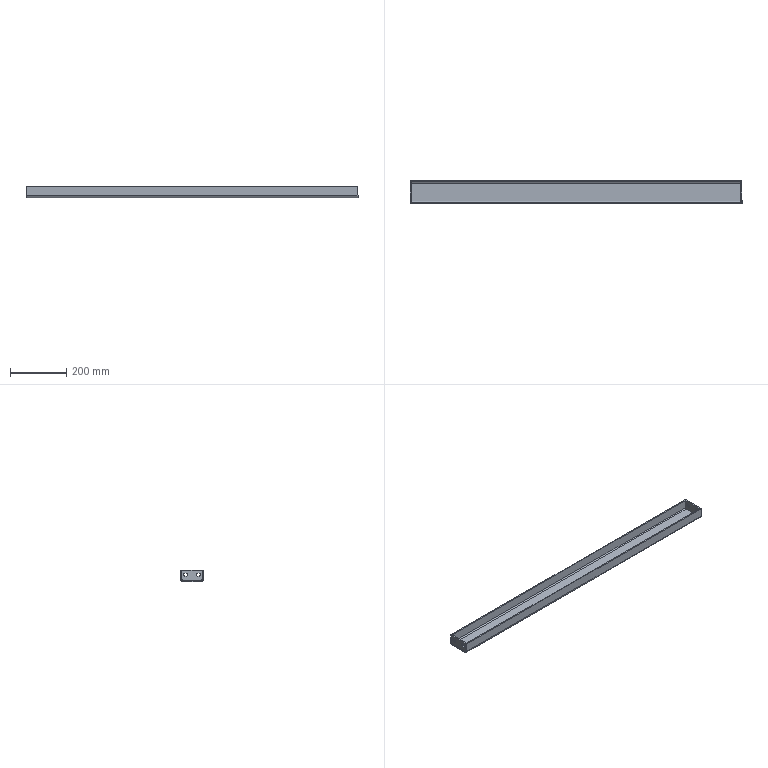Component | SolidWorks | LongitudinalStiffeningChannelSteel-1 | 3 solids | 58 faces | volume 715222 mm3 | plane 38 | cylinder 20 | commonest cylinder face diameters 11 x12 10 x4 8 x2 16 x2 | material Plain Carbon Steel